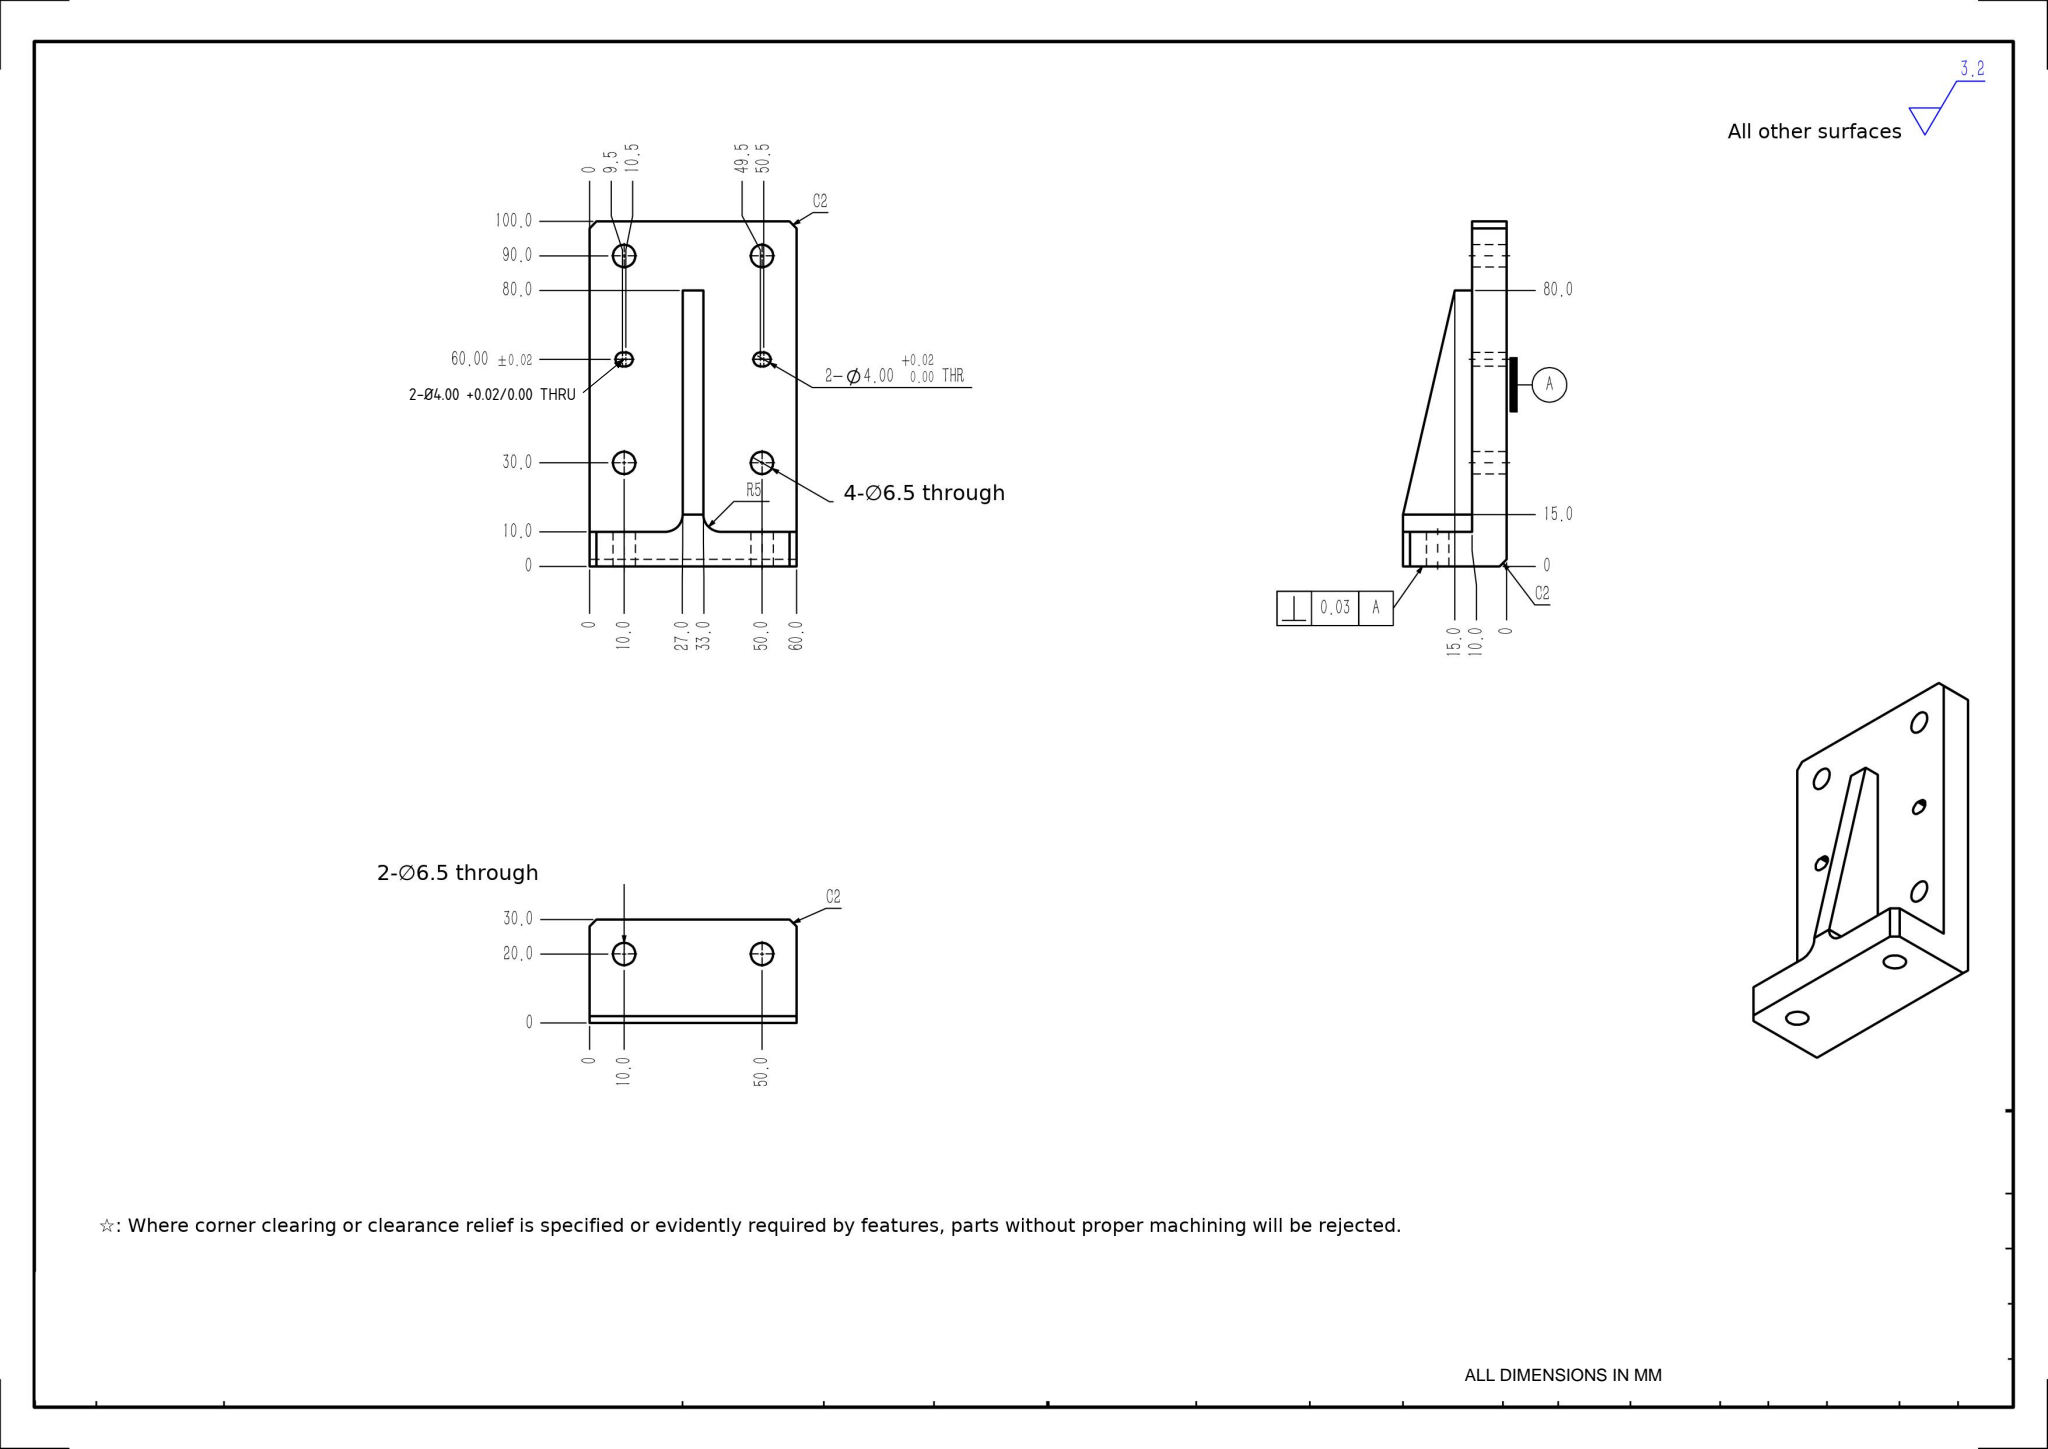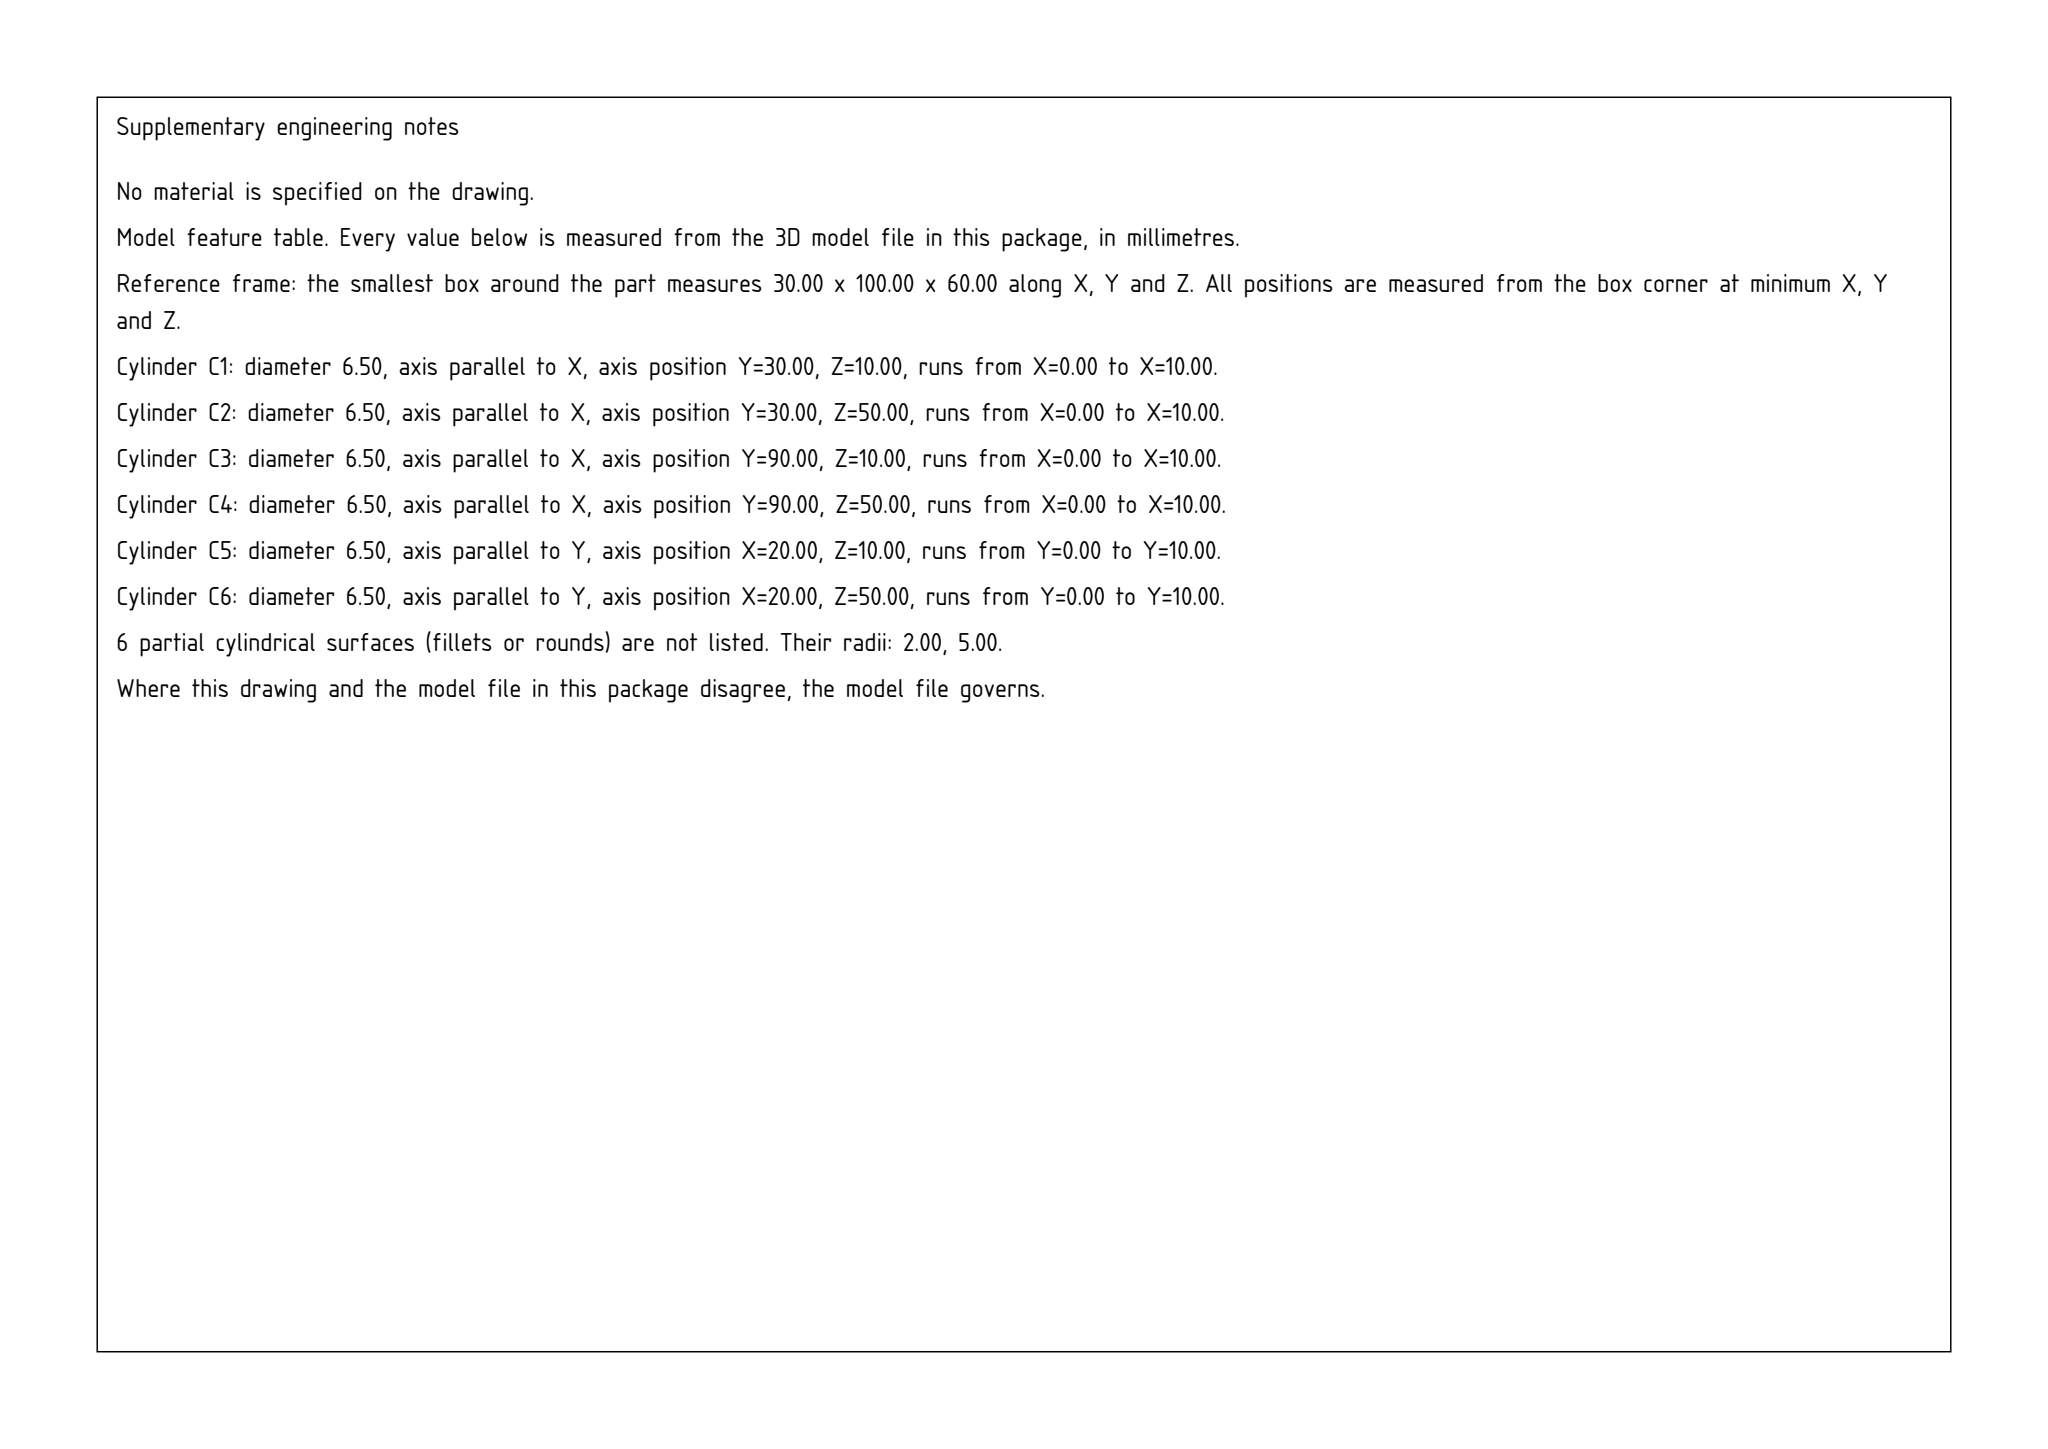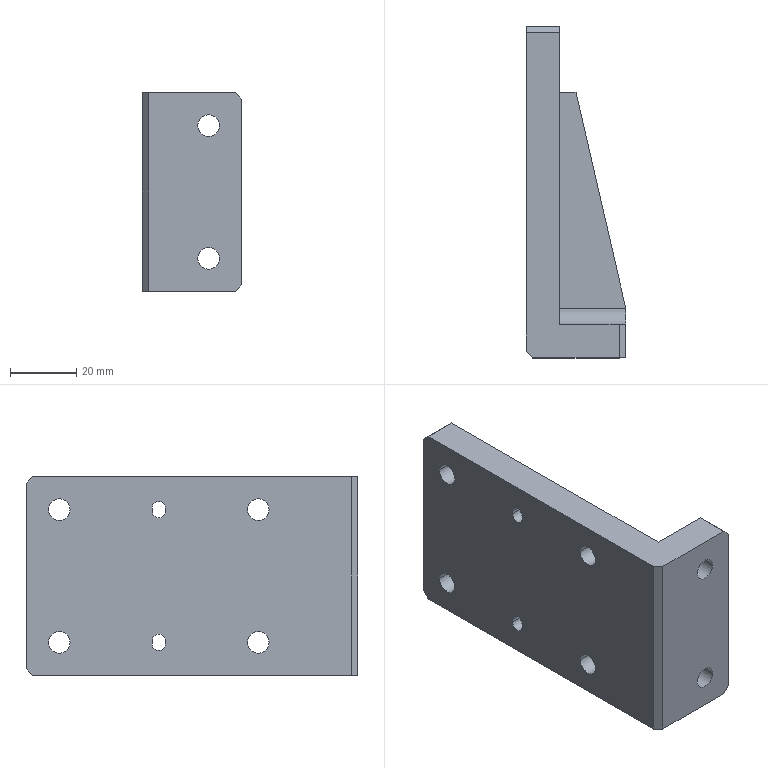Part | SolidWorks | mm | 1 solid | 40 faces | box 30 x 100 x 60 mm | volume 75167 mm3 | plane 22 | cylinder 18 | commonest cylinder face diameters 6.5 x12 4 x4 10 x2
Drawing notes:
2-Ø4.00 +0.02/0.00 THRU 10 THK VERT PLATE | from the solid: Ø4.0 cyl, axis x, len 10.0 = plate thk (x planes 0 and 10); at y60, z9.5/10.5 and z49.5/50.5
build123d program:
from build123d import *

# Parameters (mm, degrees)
BOSS_EXTRUDE1_DEPTH = 60
SKETCH2_R           = 3.25
CUT_EXTRUDE1_DEPTH  = 60
SKETCH3_R           = 3.25
CUT_EXTRUDE2_DEPTH  = 60
CUT_EXTRUDE3_DEPTH  = 119.322
CHAMFER1_SIZE       = 2
CHAMFER2_SIZE       = 2
GUSSET1_THICKNESS   = 6
FILLET1_R           = 5


with BuildPart() as part:
    # Sketch1 → Boss-Extrude1 (new body)
    with BuildSketch(Plane.XY):
        Polygon((0, 0), (0, 100), (10, 100), (10, 10), (30, 10), (30, 0), align=None)
    extrude(amount=BOSS_EXTRUDE1_DEPTH)

    # Sketch2 → Cut-Extrude1 (cut)
    with BuildSketch(Plane(origin=(0, 10, 0), x_dir=(1, 0, 0), z_dir=(0, 1, 0))):
        with Locations(Location((20, -10, 0), (0, 0, 180))):
            Circle(SKETCH2_R)
        with Locations(Location((20, -50, 0), (0, 0, 180))):
            Circle(SKETCH2_R)
    extrude(amount=-CUT_EXTRUDE1_DEPTH, mode=Mode.SUBTRACT)

    # Sketch3 → Cut-Extrude2 (cut)
    with BuildSketch(Plane(origin=(10, 0, 0), x_dir=(0, 0, -1), z_dir=(1, 0, 0))):
        with Locations(Location((-50, 30, 0), (0, 0, 90))):
            Circle(SKETCH3_R)
        with Locations((-10, 30)):
            Circle(SKETCH3_R)
        with Locations(Location((-50, 90, 0), (0, 0, 90))):
            Circle(SKETCH3_R)
        with Locations((-10, 90)):
            Circle(SKETCH3_R)
    extrude(amount=-CUT_EXTRUDE2_DEPTH, mode=Mode.SUBTRACT)

    # Sketch7 → Cut-Extrude3 (cut, through all)
    with BuildSketch(Plane(origin=(10, 0, 0), x_dir=(0, 0, -1), z_dir=(1, 0, 0))):
        with BuildLine():
            Line((-50.5, 62), (-49.5, 62))
            ThreePointArc((-49.5, 62), (-47.5, 60), (-49.5, 58))
            Line((-49.5, 58), (-50.5, 58))
            ThreePointArc((-50.5, 58), (-52.5, 60), (-50.5, 62))
        make_face()
        with BuildLine():
            Line((-9.5, 62), (-10.5, 62))
            ThreePointArc((-10.5, 62), (-12.5, 60), (-10.5, 58))
            Line((-10.5, 58), (-9.5, 58))
            ThreePointArc((-9.5, 58), (-7.5, 60), (-9.5, 62))
        make_face()
    extrude(amount=-CUT_EXTRUDE3_DEPTH, mode=Mode.SUBTRACT)

    # Chamfer1
    chamfer1_edges = [part.edges().sort_by_distance(p)[0] for p in [
        (5, 100, 60),
        (5, 100, 0),
        (30, 5, 60),
        (30, 5, 0),
    ]]
    chamfer(chamfer1_edges, length=CHAMFER1_SIZE)

    # Chamfer2
    chamfer2_edges = [part.edges().sort_by_distance(p)[0] for p in [
        (0, 0, 30),
    ]]
    chamfer(chamfer2_edges, length=CHAMFER2_SIZE)


with BuildPart() as body_2:
    # Gusset1: a gusset: a plate 6.0 thick in the corner of two members, its outline drawn in place
    gusset1_outline = Wire([Line((10, 10, 27), (10, 80, 27)), Line((10, 80, 27), (15, 80, 27)), Line((15, 80, 27), (30, 15, 27)), Line((30, 15, 27), (30, 10, 27)), Line((30, 10, 27), (10, 10, 27))])
    add(extrude(Face(gusset1_outline), amount=GUSSET1_THICKNESS, dir=(0, 0, 1)))

    # Combine1: union part
    add(part.part)

    # Fillet1
    fillet1_edges = [body_2.edges().sort_by_distance(p)[0] for p in [
        (20, 10, 27),
        (20, 10, 33),
    ]]
    fillet(fillet1_edges, radius=FILLET1_R)


solid = body_2.part